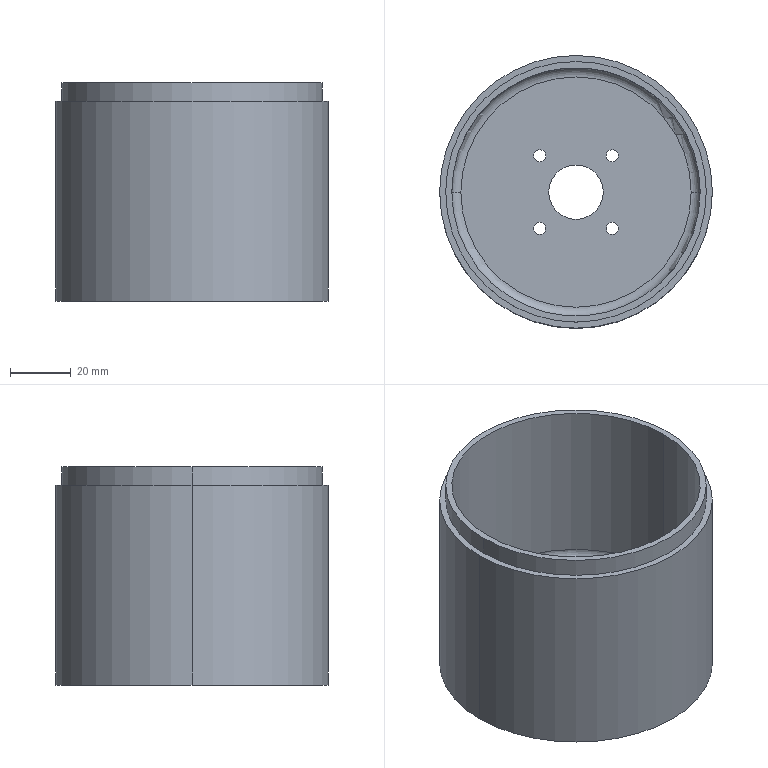Component | SolidWorks | g11-1 | 1 solid | 30 faces | box 90 x 90 x 72 mm | volume 88290 mm3 | cylinder 20 | plane 6 | torus 4 | commonest cylinder face diameters 4 x8 86 x4 82 x4 18 x2 90 x2
STEP:
#1=CARTESIAN_POINT('',(1.066,-0.06694,2.598));
#2=VERTEX_POINT('',#1);
#3=CARTESIAN_POINT('',(-2.32,-0.06694,2.598));
#4=VERTEX_POINT('',#3);
#5=CARTESIAN_POINT('',(-0.6271,-0.06694,2.598));
#6=DIRECTION('',(0.,0.,-1.));
#7=DIRECTION('',(-1.,0.,0.));
#8=AXIS2_PLACEMENT_3D('',#5,#6,#7);
#9=CIRCLE('',#8,1.693);
#10=EDGE_CURVE('',#2,#4,#9,.T.);
#11=ORIENTED_EDGE('',*,*,#10,.F.);
#12=CARTESIAN_POINT('',(1.066,-0.06694,2.441));
#13=VERTEX_POINT('',#12);
#14=CARTESIAN_POINT('',(1.066,-0.06694,2.165));
#15=DIRECTION('',(0.,0.,-1.));
#16=VECTOR('',#15,39.37);
#17=LINE('',#14,#16);
#18=EDGE_CURVE('',#2,#13,#17,.T.);
#19=ORIENTED_EDGE('',*,*,#18,.T.);
#20=CARTESIAN_POINT('',(-2.32,-0.06694,2.441));
#21=VERTEX_POINT('',#20);
#22=CARTESIAN_POINT('',(-0.6271,-0.06694,2.441));
#23=DIRECTION('',(0.,0.,-1.));
#24=DIRECTION('',(-1.,0.,0.));
#25=AXIS2_PLACEMENT_3D('',#22,#23,#24);
#26=CIRCLE('',#25,1.693);
#27=EDGE_CURVE('',#13,#21,#26,.T.);
#28=ORIENTED_EDGE('',*,*,#27,.T.);
#29=CARTESIAN_POINT('',(-2.32,-0.06694,2.165));
#30=DIRECTION('',(0.,0.,-1.));
#31=VECTOR('',#30,39.37);
#32=LINE('',#29,#31);
#33=EDGE_CURVE('',#4,#21,#32,.T.);
#34=ORIENTED_EDGE('',*,*,#33,.F.);
#35=EDGE_LOOP('',(#11,#19,#28,#34));
#36=FACE_OUTER_BOUND('',#35,.T.);
#37=CARTESIAN_POINT('',(-0.6271,-0.06694,2.165));
#38=DIRECTION('',(0.,0.,-1.));
#39=DIRECTION('',(-1.,0.,0.));
#40=AXIS2_PLACEMENT_3D('',#37,#38,#39);
#41=CYLINDRICAL_SURFACE('',#40,1.693);
#42=ADVANCED_FACE('',(#36),#41,.F.);
#43=CARTESIAN_POINT('',(-1.178,0.4055,2.992));
#44=VERTEX_POINT('',#43);
#45=CARTESIAN_POINT('',(-1.021,0.4055,2.992));
#46=VERTEX_POINT('',#45);
#47=CARTESIAN_POINT('',(-1.1,0.4055,2.992));
#48=DIRECTION('',(0.,0.,1.));
#49=DIRECTION('',(1.,0.,0.));
#50=AXIS2_PLACEMENT_3D('',#47,#48,#49);
#51=CIRCLE('',#50,0.07874);
#52=EDGE_CURVE('',#44,#46,#51,.T.);
#53=ORIENTED_EDGE('',*,*,#52,.T.);
#54=CARTESIAN_POINT('',(-1.021,0.4055,2.874));
#55=VERTEX_POINT('',#54);
#56=CARTESIAN_POINT('',(-1.021,0.4055,3.268));
#57=DIRECTION('',(0.,0.,-1.));
#58=VECTOR('',#57,39.37);
#59=LINE('',#56,#58);
#60=EDGE_CURVE('',#46,#55,#59,.T.);
#61=ORIENTED_EDGE('',*,*,#60,.T.);
#62=CARTESIAN_POINT('',(-1.178,0.4055,2.874));
#63=VERTEX_POINT('',#62);
#64=CARTESIAN_POINT('',(-1.1,0.4055,2.874));
#65=DIRECTION('',(0.,0.,-1.));
#66=DIRECTION('',(-1.,0.,0.));
#67=AXIS2_PLACEMENT_3D('',#64,#65,#66);
#68=CIRCLE('',#67,0.07874);
#69=EDGE_CURVE('',#55,#63,#68,.T.);
#70=ORIENTED_EDGE('',*,*,#69,.T.);
#71=CARTESIAN_POINT('',(-1.178,0.4055,3.268));
#72=DIRECTION('',(0.,0.,-1.));
#73=VECTOR('',#72,39.37);
#74=LINE('',#71,#73);
#75=EDGE_CURVE('',#44,#63,#74,.T.);
#76=ORIENTED_EDGE('',*,*,#75,.F.);
#77=EDGE_LOOP('',(#53,#61,#70,#76));
#78=FACE_OUTER_BOUND('',#77,.T.);
#79=CARTESIAN_POINT('',(-1.1,0.4055,3.268));
#80=DIRECTION('',(0.,0.,-1.));
#81=DIRECTION('',(-1.,0.,0.));
#82=AXIS2_PLACEMENT_3D('',#79,#80,#81);
#83=CYLINDRICAL_SURFACE('',#82,0.07874);
#84=ADVANCED_FACE('',(#78),#83,.F.);
#85=CARTESIAN_POINT('',(-0.2334,0.4055,2.992));
#86=VERTEX_POINT('',#85);
#87=CARTESIAN_POINT('',(-0.07591,0.4055,2.992));
#88=VERTEX_POINT('',#87);
#89=CARTESIAN_POINT('',(-0.1546,0.4055,2.992));
#90=DIRECTION('',(0.,0.,1.));
#91=DIRECTION('',(1.,0.,0.));
#92=AXIS2_PLACEMENT_3D('',#89,#90,#91);
#93=CIRCLE('',#92,0.07874);
#94=EDGE_CURVE('',#86,#88,#93,.T.);
#95=ORIENTED_EDGE('',*,*,#94,.T.);
#96=CARTESIAN_POINT('',(-0.07591,0.4055,2.874));
#97=VERTEX_POINT('',#96);
#98=CARTESIAN_POINT('',(-0.07591,0.4055,3.268));
#99=DIRECTION('',(0.,0.,-1.));
#100=VECTOR('',#99,39.37);
#101=LINE('',#98,#100);
#102=EDGE_CURVE('',#88,#97,#101,.T.);
#103=ORIENTED_EDGE('',*,*,#102,.T.);
#104=CARTESIAN_POINT('',(-0.2334,0.4055,2.874));
#105=VERTEX_POINT('',#104);
#106=CARTESIAN_POINT('',(-0.1546,0.4055,2.874));
#107=DIRECTION('',(0.,0.,-1.));
#108=DIRECTION('',(-1.,0.,0.));
#109=AXIS2_PLACEMENT_3D('',#106,#107,#108);
#110=CIRCLE('',#109,0.07874);
#111=EDGE_CURVE('',#97,#105,#110,.T.);
#112=ORIENTED_EDGE('',*,*,#111,.T.);
#113=CARTESIAN_POINT('',(-0.2334,0.4055,3.268));
#114=DIRECTION('',(0.,0.,-1.));
#115=VECTOR('',#114,39.37);
#116=LINE('',#113,#115);
#117=EDGE_CURVE('',#86,#105,#116,.T.);
#118=ORIENTED_EDGE('',*,*,#117,.F.);
#119=EDGE_LOOP('',(#95,#103,#112,#118));
#120=FACE_OUTER_BOUND('',#119,.T.);
#121=CARTESIAN_POINT('',(-0.1546,0.4055,3.268));
#122=DIRECTION('',(0.,0.,-1.));
#123=DIRECTION('',(-1.,0.,0.));
#124=AXIS2_PLACEMENT_3D('',#121,#122,#123);
#125=CYLINDRICAL_SURFACE('',#124,0.07874);
#126=ADVANCED_FACE('',(#120),#125,.F.);
#127=CARTESIAN_POINT('',(-0.2334,-0.5394,2.992));
#128=VERTEX_POINT('',#127);
#129=CARTESIAN_POINT('',(-0.07591,-0.5394,2.992));
#130=VERTEX_POINT('',#129);
#131=CARTESIAN_POINT('',(-0.1546,-0.5394,2.992));
#132=DIRECTION('',(0.,0.,1.));
#133=DIRECTION('',(1.,0.,0.));
#134=AXIS2_PLACEMENT_3D('',#131,#132,#133);
#135=CIRCLE('',#134,0.07874);
#136=EDGE_CURVE('',#128,#130,#135,.T.);
#137=ORIENTED_EDGE('',*,*,#136,.T.);
#138=CARTESIAN_POINT('',(-0.07591,-0.5394,2.874));
#139=VERTEX_POINT('',#138);
#140=CARTESIAN_POINT('',(-0.07591,-0.5394,3.268));
#141=DIRECTION('',(0.,0.,-1.));
#142=VECTOR('',#141,39.37);
#143=LINE('',#140,#142);
#144=EDGE_CURVE('',#130,#139,#143,.T.);
#145=ORIENTED_EDGE('',*,*,#144,.T.);
#146=CARTESIAN_POINT('',(-0.2334,-0.5394,2.874));
#147=VERTEX_POINT('',#146);
#148=CARTESIAN_POINT('',(-0.1546,-0.5394,2.874));
#149=DIRECTION('',(0.,0.,-1.));
#150=DIRECTION('',(-1.,0.,0.));
#151=AXIS2_PLACEMENT_3D('',#148,#149,#150);
#152=CIRCLE('',#151,0.07874);
#153=EDGE_CURVE('',#139,#147,#152,.T.);
#154=ORIENTED_EDGE('',*,*,#153,.T.);
#155=CARTESIAN_POINT('',(-0.2334,-0.5394,3.268));
#156=DIRECTION('',(0.,0.,-1.));
#157=VECTOR('',#156,39.37);
#158=LINE('',#155,#157);
#159=EDGE_CURVE('',#128,#147,#158,.T.);
#160=ORIENTED_EDGE('',*,*,#159,.F.);
#161=EDGE_LOOP('',(#137,#145,#154,#160));
#162=FACE_OUTER_BOUND('',#161,.T.);
#163=CARTESIAN_POINT('',(-0.1546,-0.5394,3.268));
#164=DIRECTION('',(0.,0.,-1.));
#165=DIRECTION('',(-1.,0.,0.));
#166=AXIS2_PLACEMENT_3D('',#163,#164,#165);
#167=CYLINDRICAL_SURFACE('',#166,0.07874);
#168=ADVANCED_FACE('',(#162),#167,.F.);
#169=CARTESIAN_POINT('',(-1.178,-0.5394,2.992));
#170=VERTEX_POINT('',#169);
#171=CARTESIAN_POINT('',(-1.021,-0.5394,2.992));
#172=VERTEX_POINT('',#171);
#173=CARTESIAN_POINT('',(-1.1,-0.5394,2.992));
#174=DIRECTION('',(0.,0.,1.));
#175=DIRECTION('',(1.,0.,0.));
#176=AXIS2_PLACEMENT_3D('',#173,#174,#175);
#177=CIRCLE('',#176,0.07874);
#178=EDGE_CURVE('',#170,#172,#177,.T.);
#179=ORIENTED_EDGE('',*,*,#178,.T.);
#180=CARTESIAN_POINT('',(-1.021,-0.5394,2.874));
#181=VERTEX_POINT('',#180);
#182=CARTESIAN_POINT('',(-1.021,-0.5394,3.268));
#183=DIRECTION('',(0.,0.,-1.));
#184=VECTOR('',#183,39.37);
#185=LINE('',#182,#184);
#186=EDGE_CURVE('',#172,#181,#185,.T.);
#187=ORIENTED_EDGE('',*,*,#186,.T.);
#188=CARTESIAN_POINT('',(-1.178,-0.5394,2.874));
#189=VERTEX_POINT('',#188);
#190=CARTESIAN_POINT('',(-1.1,-0.5394,2.874));
#191=DIRECTION('',(0.,0.,-1.));
#192=DIRECTION('',(-1.,0.,0.));
#193=AXIS2_PLACEMENT_3D('',#190,#191,#192);
#194=CIRCLE('',#193,0.07874);
#195=EDGE_CURVE('',#181,#189,#194,.T.);
#196=ORIENTED_EDGE('',*,*,#195,.T.);
#197=CARTESIAN_POINT('',(-1.178,-0.5394,3.268));
#198=DIRECTION('',(0.,0.,-1.));
#199=VECTOR('',#198,39.37);
#200=LINE('',#197,#199);
#201=EDGE_CURVE('',#170,#189,#200,.T.);
#202=ORIENTED_EDGE('',*,*,#201,.F.);
#203=EDGE_LOOP('',(#179,#187,#196,#202));
#204=FACE_OUTER_BOUND('',#203,.T.);
#205=CARTESIAN_POINT('',(-1.1,-0.5394,3.268));
#206=DIRECTION('',(0.,0.,-1.));
#207=DIRECTION('',(-1.,0.,0.));
#208=AXIS2_PLACEMENT_3D('',#205,#206,#207);
#209=CYLINDRICAL_SURFACE('',#208,0.07874);
#210=ADVANCED_FACE('',(#204),#209,.F.);
#211=CARTESIAN_POINT('',(0.869,-0.06694,2.874));
#212=VERTEX_POINT('',#211);
#213=CARTESIAN_POINT('',(-2.123,-0.06694,2.874));
#214=VERTEX_POINT('',#213);
#215=CARTESIAN_POINT('',(-0.6271,-0.06694,2.874));
#216=DIRECTION('',(0.,0.,-1.));
#217=DIRECTION('',(-1.,0.,0.));
#218=AXIS2_PLACEMENT_3D('',#215,#216,#217);
#219=CIRCLE('',#218,1.496);
#220=EDGE_CURVE('',#212,#214,#219,.T.);
#221=ORIENTED_EDGE('',*,*,#220,.F.);
#222=CARTESIAN_POINT('',(0.9871,-0.06694,2.756));
#223=VERTEX_POINT('',#222);
#224=CARTESIAN_POINT('',(0.869,-0.06694,2.756));
#225=DIRECTION('',(-0.,1.,0.));
#226=DIRECTION('',(-1.,-0.,0.));
#227=AXIS2_PLACEMENT_3D('',#224,#225,#226);
#228=CIRCLE('',#227,0.1181);
#229=EDGE_CURVE('',#212,#223,#228,.T.);
#230=ORIENTED_EDGE('',*,*,#229,.T.);
#231=CARTESIAN_POINT('',(-2.241,-0.06694,2.756));
#232=VERTEX_POINT('',#231);
#233=CARTESIAN_POINT('',(-0.6271,-0.06694,2.756));
#234=DIRECTION('',(0.,0.,1.));
#235=DIRECTION('',(-1.,0.,0.));
#236=AXIS2_PLACEMENT_3D('',#233,#234,#235);
#237=CIRCLE('',#236,1.614);
#238=EDGE_CURVE('',#232,#223,#237,.T.);
#239=ORIENTED_EDGE('',*,*,#238,.F.);
#240=CARTESIAN_POINT('',(-2.123,-0.06694,2.756));
#241=DIRECTION('',(0.,-1.,0.));
#242=DIRECTION('',(0.,0.,-1.));
#243=AXIS2_PLACEMENT_3D('',#240,#241,#242);
#244=CIRCLE('',#243,0.1181);
#245=EDGE_CURVE('',#214,#232,#244,.T.);
#246=ORIENTED_EDGE('',*,*,#245,.F.);
#247=EDGE_LOOP('',(#221,#230,#239,#246));
#248=FACE_OUTER_BOUND('',#247,.T.);
#249=CARTESIAN_POINT('',(-0.6271,-0.06694,2.756));
#250=DIRECTION('',(0.,0.,-1.));
#251=DIRECTION('',(-1.,0.,0.));
#252=AXIS2_PLACEMENT_3D('',#249,#250,#251);
#253=TOROIDAL_SURFACE('',#252,1.496,0.1181);
#254=ADVANCED_FACE('',(#248),#253,.F.);
#255=CARTESIAN_POINT('',(-2.123,-0.06694,2.992));
#256=VERTEX_POINT('',#255);
#257=CARTESIAN_POINT('',(0.869,-0.06694,2.992));
#258=VERTEX_POINT('',#257);
#259=CARTESIAN_POINT('',(-0.6271,-0.06694,2.992));
#260=DIRECTION('',(0.,0.,1.));
#261=DIRECTION('',(1.,0.,0.));
#262=AXIS2_PLACEMENT_3D('',#259,#260,#261);
#263=CIRCLE('',#262,1.496);
#264=EDGE_CURVE('',#256,#258,#263,.T.);
#265=ORIENTED_EDGE('',*,*,#264,.F.);
#266=CARTESIAN_POINT('',(-2.241,-0.06694,3.11));
#267=VERTEX_POINT('',#266);
#268=CARTESIAN_POINT('',(-2.123,-0.06694,3.11));
#269=DIRECTION('',(0.,1.,0.));
#270=DIRECTION('',(-1.,0.,0.));
#271=AXIS2_PLACEMENT_3D('',#268,#269,#270);
#272=CIRCLE('',#271,0.1181);
#273=EDGE_CURVE('',#256,#267,#272,.T.);
#274=ORIENTED_EDGE('',*,*,#273,.T.);
#275=CARTESIAN_POINT('',(0.9871,-0.06694,3.11));
#276=VERTEX_POINT('',#275);
#277=CARTESIAN_POINT('',(-0.6271,-0.06694,3.11));
#278=DIRECTION('',(0.,0.,-1.));
#279=DIRECTION('',(1.,0.,0.));
#280=AXIS2_PLACEMENT_3D('',#277,#278,#279);
#281=CIRCLE('',#280,1.614);
#282=EDGE_CURVE('',#276,#267,#281,.T.);
#283=ORIENTED_EDGE('',*,*,#282,.F.);
#284=CARTESIAN_POINT('',(0.869,-0.06694,3.11));
#285=DIRECTION('',(0.,-1.,0.));
#286=DIRECTION('',(0.,0.,-1.));
#287=AXIS2_PLACEMENT_3D('',#284,#285,#286);
#288=CIRCLE('',#287,0.1181);
#289=EDGE_CURVE('',#258,#276,#288,.T.);
#290=ORIENTED_EDGE('',*,*,#289,.F.);
#291=EDGE_LOOP('',(#265,#274,#283,#290));
#292=FACE_OUTER_BOUND('',#291,.T.);
#293=CARTESIAN_POINT('',(-0.6271,-0.06694,3.11));
#294=DIRECTION('',(0.,0.,1.));
#295=DIRECTION('',(1.,0.,0.));
#296=AXIS2_PLACEMENT_3D('',#293,#294,#295);
#297=TOROIDAL_SURFACE('',#296,1.496,0.1181);
#298=ADVANCED_FACE('',(#292),#297,.F.);
#299=CARTESIAN_POINT('',(-0.2728,-0.06694,2.992));
#300=VERTEX_POINT('',#299);
#301=CARTESIAN_POINT('',(-0.9814,-0.06694,2.992));
#302=VERTEX_POINT('',#301);
#303=CARTESIAN_POINT('',(-0.6271,-0.06694,2.992));
#304=DIRECTION('',(0.,0.,-1.));
#305=DIRECTION('',(-1.,0.,0.));
#306=AXIS2_PLACEMENT_3D('',#303,#304,#305);
#307=CIRCLE('',#306,0.3543);
#308=EDGE_CURVE('',#300,#302,#307,.T.);
#309=ORIENTED_EDGE('',*,*,#308,.F.);
#310=CARTESIAN_POINT('',(-0.2728,-0.06694,2.874));
#311=VERTEX_POINT('',#310);
#312=CARTESIAN_POINT('',(-0.2728,-0.06694,2.441));
#313=DIRECTION('',(0.,0.,-1.));
#314=VECTOR('',#313,39.37);
#315=LINE('',#312,#314);
#316=EDGE_CURVE('',#300,#311,#315,.T.);
#317=ORIENTED_EDGE('',*,*,#316,.T.);
#318=CARTESIAN_POINT('',(-0.9814,-0.06694,2.874));
#319=VERTEX_POINT('',#318);
#320=CARTESIAN_POINT('',(-0.6271,-0.06694,2.874));
#321=DIRECTION('',(0.,0.,-1.));
#322=DIRECTION('',(-1.,0.,0.));
#323=AXIS2_PLACEMENT_3D('',#320,#321,#322);
#324=CIRCLE('',#323,0.3543);
#325=EDGE_CURVE('',#311,#319,#324,.T.);
#326=ORIENTED_EDGE('',*,*,#325,.T.);
#327=CARTESIAN_POINT('',(-0.9814,-0.06694,2.441));
#328=DIRECTION('',(0.,0.,-1.));
#329=VECTOR('',#328,39.37);
#330=LINE('',#327,#329);
#331=EDGE_CURVE('',#302,#319,#330,.T.);
#332=ORIENTED_EDGE('',*,*,#331,.F.);
#333=EDGE_LOOP('',(#309,#317,#326,#332));
#334=FACE_OUTER_BOUND('',#333,.T.);
#335=CARTESIAN_POINT('',(-0.6271,-0.06694,2.441));
#336=DIRECTION('',(0.,0.,-1.));
#337=DIRECTION('',(-1.,0.,0.));
#338=AXIS2_PLACEMENT_3D('',#335,#336,#337);
#339=CYLINDRICAL_SURFACE('',#338,0.3543);
#340=ADVANCED_FACE('',(#334),#339,.F.);
#341=CARTESIAN_POINT('',(-2.32,-0.06694,5.276));
#342=VERTEX_POINT('',#341);
#343=CARTESIAN_POINT('',(1.066,-0.06694,5.276));
#344=VERTEX_POINT('',#343);
#345=CARTESIAN_POINT('',(-0.6271,-0.06694,5.276));
#346=DIRECTION('',(0.,0.,-1.));
#347=DIRECTION('',(-1.,0.,0.));
#348=AXIS2_PLACEMENT_3D('',#345,#346,#347);
#349=CIRCLE('',#348,1.693);
#350=EDGE_CURVE('',#342,#344,#349,.T.);
#351=ORIENTED_EDGE('',*,*,#350,.T.);
#352=CARTESIAN_POINT('',(1.066,-0.06694,5.039));
#353=VERTEX_POINT('',#352);
#354=CARTESIAN_POINT('',(1.066,-0.06694,5.276));
#355=DIRECTION('',(0.,0.,-1.));
#356=VECTOR('',#355,39.37);
#357=LINE('',#354,#356);
#358=EDGE_CURVE('',#344,#353,#357,.T.);
#359=ORIENTED_EDGE('',*,*,#358,.T.);
#360=CARTESIAN_POINT('',(-2.32,-0.06694,5.039));
#361=VERTEX_POINT('',#360);
#362=CARTESIAN_POINT('',(-0.6271,-0.06694,5.039));
#363=DIRECTION('',(0.,0.,1.));
#364=DIRECTION('',(1.,0.,0.));
#365=AXIS2_PLACEMENT_3D('',#362,#363,#364);
#366=CIRCLE('',#365,1.693);
#367=EDGE_CURVE('',#353,#361,#366,.T.);
#368=ORIENTED_EDGE('',*,*,#367,.T.);
#369=CARTESIAN_POINT('',(-2.32,-0.06694,5.276));
#370=DIRECTION('',(0.,0.,-1.));
#371=VECTOR('',#370,39.37);
#372=LINE('',#369,#371);
#373=EDGE_CURVE('',#342,#361,#372,.T.);
#374=ORIENTED_EDGE('',*,*,#373,.F.);
#375=EDGE_LOOP('',(#351,#359,#368,#374));
#376=FACE_OUTER_BOUND('',#375,.T.);
#377=CARTESIAN_POINT('',(-0.6271,-0.06694,5.276));
#378=DIRECTION('',(0.,0.,-1.));
#379=DIRECTION('',(-1.,0.,0.));
#380=AXIS2_PLACEMENT_3D('',#377,#378,#379);
#381=CYLINDRICAL_SURFACE('',#380,1.693);
#382=ADVANCED_FACE('',(#376),#381,.T.);
#383=ORIENTED_EDGE('',*,*,#238,.T.);
#384=CARTESIAN_POINT('',(0.9871,-0.06694,2.598));
#385=VERTEX_POINT('',#384);
#386=CARTESIAN_POINT('',(0.9871,-0.06694,5.039));
#387=DIRECTION('',(0.,0.,-1.));
#388=VECTOR('',#387,39.37);
#389=LINE('',#386,#388);
#390=EDGE_CURVE('',#223,#385,#389,.T.);
#391=ORIENTED_EDGE('',*,*,#390,.T.);
#392=CARTESIAN_POINT('',(-2.241,-0.06694,2.598));
#393=VERTEX_POINT('',#392);
#394=CARTESIAN_POINT('',(-0.6271,-0.06694,2.598));
#395=DIRECTION('',(0.,0.,1.));
#396=DIRECTION('',(1.,0.,0.));
#397=AXIS2_PLACEMENT_3D('',#394,#395,#396);
#398=CIRCLE('',#397,1.614);
#399=EDGE_CURVE('',#393,#385,#398,.T.);
#400=ORIENTED_EDGE('',*,*,#399,.F.);
#401=CARTESIAN_POINT('',(-2.241,-0.06694,5.039));
#402=DIRECTION('',(0.,0.,-1.));
#403=VECTOR('',#402,39.37);
#404=LINE('',#401,#403);
#405=EDGE_CURVE('',#232,#393,#404,.T.);
#406=ORIENTED_EDGE('',*,*,#405,.F.);
#407=EDGE_LOOP('',(#383,#391,#400,#406));
#408=FACE_OUTER_BOUND('',#407,.T.);
#409=CARTESIAN_POINT('',(-0.6271,-0.06694,5.039));
#410=DIRECTION('',(0.,0.,-1.));
#411=DIRECTION('',(-1.,0.,0.));
#412=AXIS2_PLACEMENT_3D('',#409,#410,#411);
#413=CYLINDRICAL_SURFACE('',#412,1.614);
#414=ADVANCED_FACE('',(#408),#413,.F.);
#415=CARTESIAN_POINT('',(1.145,-0.06694,5.039));
#416=VERTEX_POINT('',#415);
#417=CARTESIAN_POINT('',(-2.399,-0.06694,5.039));
#418=VERTEX_POINT('',#417);
#419=CARTESIAN_POINT('',(-0.6271,-0.06694,5.039));
#420=DIRECTION('',(0.,0.,1.));
#421=DIRECTION('',(1.,0.,0.));
#422=AXIS2_PLACEMENT_3D('',#419,#420,#421);
#423=CIRCLE('',#422,1.772);
#424=EDGE_CURVE('',#416,#418,#423,.T.);
#425=ORIENTED_EDGE('',*,*,#424,.F.);
#426=CARTESIAN_POINT('',(1.145,-0.06694,2.441));
#427=VERTEX_POINT('',#426);
#428=CARTESIAN_POINT('',(1.145,-0.06694,5.039));
#429=DIRECTION('',(0.,0.,-1.));
#430=VECTOR('',#429,39.37);
#431=LINE('',#428,#430);
#432=EDGE_CURVE('',#416,#427,#431,.T.);
#433=ORIENTED_EDGE('',*,*,#432,.T.);
#434=CARTESIAN_POINT('',(-2.399,-0.06694,2.441));
#435=VERTEX_POINT('',#434);
#436=CARTESIAN_POINT('',(-0.6271,-0.06694,2.441));
#437=DIRECTION('',(0.,0.,-1.));
#438=DIRECTION('',(-1.,0.,0.));
#439=AXIS2_PLACEMENT_3D('',#436,#437,#438);
#440=CIRCLE('',#439,1.772);
#441=EDGE_CURVE('',#435,#427,#440,.T.);
#442=ORIENTED_EDGE('',*,*,#441,.F.);
#443=CARTESIAN_POINT('',(-2.399,-0.06694,5.039));
#444=DIRECTION('',(0.,0.,-1.));
#445=VECTOR('',#444,39.37);
#446=LINE('',#443,#445);
#447=EDGE_CURVE('',#418,#435,#446,.T.);
#448=ORIENTED_EDGE('',*,*,#447,.F.);
#449=EDGE_LOOP('',(#425,#433,#442,#448));
#450=FACE_OUTER_BOUND('',#449,.T.);
#451=CARTESIAN_POINT('',(-0.6271,-0.06694,5.039));
#452=DIRECTION('',(0.,0.,-1.));
#453=DIRECTION('',(-1.,0.,0.));
#454=AXIS2_PLACEMENT_3D('',#451,#452,#453);
#455=CYLINDRICAL_SURFACE('',#454,1.772);
#456=ADVANCED_FACE('',(#450),#455,.T.);
#457=CARTESIAN_POINT('',(0.9871,-0.06694,5.276));
#458=VERTEX_POINT('',#457);
#459=CARTESIAN_POINT('',(-2.241,-0.06694,5.276));
#460=VERTEX_POINT('',#459);
#461=CARTESIAN_POINT('',(-0.6271,-0.06694,5.276));
#462=DIRECTION('',(0.,0.,-1.));
#463=DIRECTION('',(-1.,0.,0.));
#464=AXIS2_PLACEMENT_3D('',#461,#462,#463);
#465=CIRCLE('',#464,1.614);
#466=EDGE_CURVE('',#458,#460,#465,.T.);
#467=ORIENTED_EDGE('',*,*,#466,.F.);
#468=CARTESIAN_POINT('',(0.9871,-0.06694,5.039));
#469=DIRECTION('',(0.,0.,-1.));
#470=VECTOR('',#469,39.37);
#471=LINE('',#468,#470);
#472=EDGE_CURVE('',#458,#276,#471,.T.);
#473=ORIENTED_EDGE('',*,*,#472,.T.);
#474=ORIENTED_EDGE('',*,*,#282,.T.);
#475=CARTESIAN_POINT('',(-2.241,-0.06694,5.039));
#476=DIRECTION('',(0.,0.,-1.));
#477=VECTOR('',#476,39.37);
#478=LINE('',#475,#477);
#479=EDGE_CURVE('',#460,#267,#478,.T.);
#480=ORIENTED_EDGE('',*,*,#479,.F.);
#481=EDGE_LOOP('',(#467,#473,#474,#480));
#482=FACE_OUTER_BOUND('',#481,.T.);
#483=CARTESIAN_POINT('',(-0.6271,-0.06694,5.039));
#484=DIRECTION('',(0.,0.,-1.));
#485=DIRECTION('',(-1.,0.,0.));
#486=AXIS2_PLACEMENT_3D('',#483,#484,#485);
#487=CYLINDRICAL_SURFACE('',#486,1.614);
#488=ADVANCED_FACE('',(#482),#487,.F.);
#489=ORIENTED_EDGE('',*,*,#472,.F.);
#490=CARTESIAN_POINT('',(-0.6271,-0.06694,5.276));
#491=DIRECTION('',(0.,0.,-1.));
#492=DIRECTION('',(-1.,0.,0.));
#493=AXIS2_PLACEMENT_3D('',#490,#491,#492);
#494=CIRCLE('',#493,1.614);
#495=EDGE_CURVE('',#460,#458,#494,.T.);
#496=ORIENTED_EDGE('',*,*,#495,.F.);
#497=ORIENTED_EDGE('',*,*,#479,.T.);
#498=CARTESIAN_POINT('',(-0.6271,-0.06694,3.11));
#499=DIRECTION('',(0.,0.,-1.));
#500=DIRECTION('',(1.,0.,0.));
#501=AXIS2_PLACEMENT_3D('',#498,#499,#500);
#502=CIRCLE('',#501,1.614);
#503=EDGE_CURVE('',#267,#276,#502,.T.);
#504=ORIENTED_EDGE('',*,*,#503,.T.);
#505=EDGE_LOOP('',(#489,#496,#497,#504));
#506=FACE_OUTER_BOUND('',#505,.T.);
#507=CARTESIAN_POINT('',(-0.6271,-0.06694,5.039));
#508=DIRECTION('',(0.,0.,-1.));
#509=DIRECTION('',(-1.,0.,0.));
#510=AXIS2_PLACEMENT_3D('',#507,#508,#509);
#511=CYLINDRICAL_SURFACE('',#510,1.614);
#512=ADVANCED_FACE('',(#506),#511,.F.);
#513=CARTESIAN_POINT('',(-0.6271,-0.06694,5.039));
#514=DIRECTION('',(0.,0.,1.));
#515=DIRECTION('',(1.,0.,0.));
#516=AXIS2_PLACEMENT_3D('',#513,#514,#515);
#517=CIRCLE('',#516,1.693);
#518=EDGE_CURVE('',#361,#353,#517,.T.);
#519=ORIENTED_EDGE('',*,*,#518,.F.);
#520=ORIENTED_EDGE('',*,*,#367,.F.);
#521=EDGE_LOOP('',(#519,#520));
#522=FACE_BOUND('',#521,.T.);
#523=CARTESIAN_POINT('',(-0.6271,-0.06694,5.039));
#524=DIRECTION('',(0.,0.,1.));
#525=DIRECTION('',(1.,0.,0.));
#526=AXIS2_PLACEMENT_3D('',#523,#524,#525);
#527=CIRCLE('',#526,1.772);
#528=EDGE_CURVE('',#418,#416,#527,.T.);
#529=ORIENTED_EDGE('',*,*,#528,.T.);
#530=ORIENTED_EDGE('',*,*,#424,.T.);
#531=EDGE_LOOP('',(#529,#530));
#532=FACE_OUTER_BOUND('',#531,.T.);
#533=CARTESIAN_POINT('',(-0.6271,-0.06694,5.039));
#534=DIRECTION('',(0.,0.,1.));
#535=DIRECTION('',(1.,0.,0.));
#536=AXIS2_PLACEMENT_3D('',#533,#534,#535);
#537=PLANE('',#536);
#538=ADVANCED_FACE('',(#522,#532),#537,.T.);
#539=ORIENTED_EDGE('',*,*,#432,.F.);
#540=ORIENTED_EDGE('',*,*,#528,.F.);
#541=ORIENTED_EDGE('',*,*,#447,.T.);
#542=CARTESIAN_POINT('',(-0.6271,-0.06694,2.441));
#543=DIRECTION('',(0.,0.,-1.));
#544=DIRECTION('',(-1.,0.,0.));
#545=AXIS2_PLACEMENT_3D('',#542,#543,#544);
#546=CIRCLE('',#545,1.772);
#547=EDGE_CURVE('',#427,#435,#546,.T.);
#548=ORIENTED_EDGE('',*,*,#547,.F.);
#549=EDGE_LOOP('',(#539,#540,#541,#548));
#550=FACE_OUTER_BOUND('',#549,.T.);
#551=CARTESIAN_POINT('',(-0.6271,-0.06694,5.039));
#552=DIRECTION('',(0.,0.,-1.));
#553=DIRECTION('',(-1.,0.,0.));
#554=AXIS2_PLACEMENT_3D('',#551,#552,#553);
#555=CYLINDRICAL_SURFACE('',#554,1.772);
#556=ADVANCED_FACE('',(#550),#555,.T.);
#557=ORIENTED_EDGE('',*,*,#390,.F.);
#558=CARTESIAN_POINT('',(-0.6271,-0.06694,2.756));
#559=DIRECTION('',(0.,0.,1.));
#560=DIRECTION('',(-1.,0.,0.));
#561=AXIS2_PLACEMENT_3D('',#558,#559,#560);
#562=CIRCLE('',#561,1.614);
#563=EDGE_CURVE('',#223,#232,#562,.T.);
#564=ORIENTED_EDGE('',*,*,#563,.T.);
#565=ORIENTED_EDGE('',*,*,#405,.T.);
#566=CARTESIAN_POINT('',(-0.6271,-0.06694,2.598));
#567=DIRECTION('',(0.,0.,1.));
#568=DIRECTION('',(1.,0.,0.));
#569=AXIS2_PLACEMENT_3D('',#566,#567,#568);
#570=CIRCLE('',#569,1.614);
#571=EDGE_CURVE('',#385,#393,#570,.T.);
#572=ORIENTED_EDGE('',*,*,#571,.F.);
#573=EDGE_LOOP('',(#557,#564,#565,#572));
#574=FACE_OUTER_BOUND('',#573,.T.);
#575=CARTESIAN_POINT('',(-0.6271,-0.06694,5.039));
#576=DIRECTION('',(0.,0.,-1.));
#577=DIRECTION('',(-1.,0.,0.));
#578=AXIS2_PLACEMENT_3D('',#575,#576,#577);
#579=CYLINDRICAL_SURFACE('',#578,1.614);
#580=ADVANCED_FACE('',(#574),#579,.F.);
#581=CARTESIAN_POINT('',(-0.6271,-0.06694,2.441));
#582=DIRECTION('',(0.,0.,-1.));
#583=DIRECTION('',(-1.,0.,0.));
#584=AXIS2_PLACEMENT_3D('',#581,#582,#583);
#585=CIRCLE('',#584,1.693);
#586=EDGE_CURVE('',#21,#13,#585,.T.);
#587=ORIENTED_EDGE('',*,*,#586,.F.);
#588=ORIENTED_EDGE('',*,*,#27,.F.);
#589=EDGE_LOOP('',(#587,#588));
#590=FACE_BOUND('',#589,.T.);
#591=ORIENTED_EDGE('',*,*,#441,.T.);
#592=ORIENTED_EDGE('',*,*,#547,.T.);
#593=EDGE_LOOP('',(#591,#592));
#594=FACE_OUTER_BOUND('',#593,.T.);
#595=CARTESIAN_POINT('',(-0.6271,-0.06694,2.441));
#596=DIRECTION('',(0.,0.,-1.));
#597=DIRECTION('',(-1.,0.,0.));
#598=AXIS2_PLACEMENT_3D('',#595,#596,#597);
#599=PLANE('',#598);
#600=ADVANCED_FACE('',(#590,#594),#599,.T.);
#601=ORIENTED_EDGE('',*,*,#358,.F.);
#602=CARTESIAN_POINT('',(-0.6271,-0.06694,5.276));
#603=DIRECTION('',(0.,0.,-1.));
#604=DIRECTION('',(-1.,0.,0.));
#605=AXIS2_PLACEMENT_3D('',#602,#603,#604);
#606=CIRCLE('',#605,1.693);
#607=EDGE_CURVE('',#344,#342,#606,.T.);
#608=ORIENTED_EDGE('',*,*,#607,.T.);
#609=ORIENTED_EDGE('',*,*,#373,.T.);
#610=ORIENTED_EDGE('',*,*,#518,.T.);
#611=EDGE_LOOP('',(#601,#608,#609,#610));
#612=FACE_OUTER_BOUND('',#611,.T.);
#613=CARTESIAN_POINT('',(-0.6271,-0.06694,5.276));
#614=DIRECTION('',(0.,0.,-1.));
#615=DIRECTION('',(-1.,0.,0.));
#616=AXIS2_PLACEMENT_3D('',#613,#614,#615);
#617=CYLINDRICAL_SURFACE('',#616,1.693);
#618=ADVANCED_FACE('',(#612),#617,.T.);
#619=ORIENTED_EDGE('',*,*,#495,.T.);
#620=ORIENTED_EDGE('',*,*,#466,.T.);
#621=EDGE_LOOP('',(#619,#620));
#622=FACE_BOUND('',#621,.T.);
#623=ORIENTED_EDGE('',*,*,#350,.F.);
#624=ORIENTED_EDGE('',*,*,#607,.F.);
#625=EDGE_LOOP('',(#623,#624));
#626=FACE_OUTER_BOUND('',#625,.T.);
#627=CARTESIAN_POINT('',(-0.6271,-0.06694,5.276));
#628=DIRECTION('',(0.,0.,1.));
#629=DIRECTION('',(-1.,0.,0.));
#630=AXIS2_PLACEMENT_3D('',#627,#628,#629);
#631=PLANE('',#630);
#632=ADVANCED_FACE('',(#622,#626),#631,.T.);
#633=ORIENTED_EDGE('',*,*,#52,.F.);
#634=CARTESIAN_POINT('',(-1.1,0.4055,2.992));
#635=DIRECTION('',(0.,0.,1.));
#636=DIRECTION('',(1.,0.,0.));
#637=AXIS2_PLACEMENT_3D('',#634,#635,#636);
#638=CIRCLE('',#637,0.07874);
#639=EDGE_CURVE('',#46,#44,#638,.T.);
#640=ORIENTED_EDGE('',*,*,#639,.F.);
#641=EDGE_LOOP('',(#633,#640));
#642=FACE_BOUND('',#641,.T.);
#643=ORIENTED_EDGE('',*,*,#94,.F.);
#644=CARTESIAN_POINT('',(-0.1546,0.4055,2.992));
#645=DIRECTION('',(0.,0.,1.));
#646=DIRECTION('',(1.,0.,0.));
#647=AXIS2_PLACEMENT_3D('',#644,#645,#646);
#648=CIRCLE('',#647,0.07874);
#649=EDGE_CURVE('',#88,#86,#648,.T.);
#650=ORIENTED_EDGE('',*,*,#649,.F.);
#651=EDGE_LOOP('',(#643,#650));
#652=FACE_BOUND('',#651,.T.);
#653=ORIENTED_EDGE('',*,*,#136,.F.);
#654=CARTESIAN_POINT('',(-0.1546,-0.5394,2.992));
#655=DIRECTION('',(0.,0.,1.));
#656=DIRECTION('',(1.,0.,0.));
#657=AXIS2_PLACEMENT_3D('',#654,#655,#656);
#658=CIRCLE('',#657,0.07874);
#659=EDGE_CURVE('',#130,#128,#658,.T.);
#660=ORIENTED_EDGE('',*,*,#659,.F.);
#661=EDGE_LOOP('',(#653,#660));
#662=FACE_BOUND('',#661,.T.);
#663=ORIENTED_EDGE('',*,*,#178,.F.);
#664=CARTESIAN_POINT('',(-1.1,-0.5394,2.992));
#665=DIRECTION('',(0.,0.,1.));
#666=DIRECTION('',(1.,0.,0.));
#667=AXIS2_PLACEMENT_3D('',#664,#665,#666);
#668=CIRCLE('',#667,0.07874);
#669=EDGE_CURVE('',#172,#170,#668,.T.);
#670=ORIENTED_EDGE('',*,*,#669,.F.);
#671=EDGE_LOOP('',(#663,#670));
#672=FACE_BOUND('',#671,.T.);
#673=CARTESIAN_POINT('',(-0.6271,-0.06694,2.992));
#674=DIRECTION('',(0.,0.,1.));
#675=DIRECTION('',(1.,0.,0.));
#676=AXIS2_PLACEMENT_3D('',#673,#674,#675);
#677=CIRCLE('',#676,1.496);
#678=EDGE_CURVE('',#258,#256,#677,.T.);
#679=ORIENTED_EDGE('',*,*,#678,.T.);
#680=ORIENTED_EDGE('',*,*,#264,.T.);
#681=EDGE_LOOP('',(#679,#680));
#682=FACE_OUTER_BOUND('',#681,.T.);
#683=CARTESIAN_POINT('',(-0.6271,-0.06694,2.992));
#684=DIRECTION('',(0.,0.,-1.));
#685=DIRECTION('',(-1.,0.,0.));
#686=AXIS2_PLACEMENT_3D('',#683,#684,#685);
#687=CIRCLE('',#686,0.3543);
#688=EDGE_CURVE('',#302,#300,#687,.T.);
#689=ORIENTED_EDGE('',*,*,#688,.T.);
#690=ORIENTED_EDGE('',*,*,#308,.T.);
#691=EDGE_LOOP('',(#689,#690));
#692=FACE_BOUND('',#691,.T.);
#693=CARTESIAN_POINT('',(-2.399,-0.06694,2.992));
#694=DIRECTION('',(0.,0.,1.));
#695=DIRECTION('',(1.,0.,0.));
#696=AXIS2_PLACEMENT_3D('',#693,#694,#695);
#697=PLANE('',#696);
#698=ADVANCED_FACE('',(#642,#652,#662,#672,#682,#692),#697,.T.);
#699=ORIENTED_EDGE('',*,*,#316,.F.);
#700=ORIENTED_EDGE('',*,*,#688,.F.);
#701=ORIENTED_EDGE('',*,*,#331,.T.);
#702=CARTESIAN_POINT('',(-0.6271,-0.06694,2.874));
#703=DIRECTION('',(0.,0.,-1.));
#704=DIRECTION('',(-1.,0.,0.));
#705=AXIS2_PLACEMENT_3D('',#702,#703,#704);
#706=CIRCLE('',#705,0.3543);
#707=EDGE_CURVE('',#319,#311,#706,.T.);
#708=ORIENTED_EDGE('',*,*,#707,.T.);
#709=EDGE_LOOP('',(#699,#700,#701,#708));
#710=FACE_OUTER_BOUND('',#709,.T.);
#711=CARTESIAN_POINT('',(-0.6271,-0.06694,2.441));
#712=DIRECTION('',(0.,0.,-1.));
#713=DIRECTION('',(-1.,0.,0.));
#714=AXIS2_PLACEMENT_3D('',#711,#712,#713);
#715=CYLINDRICAL_SURFACE('',#714,0.3543);
#716=ADVANCED_FACE('',(#710),#715,.F.);
#717=CARTESIAN_POINT('',(-1.1,0.4055,2.874));
#718=DIRECTION('',(0.,0.,-1.));
#719=DIRECTION('',(-1.,0.,0.));
#720=AXIS2_PLACEMENT_3D('',#717,#718,#719);
#721=CIRCLE('',#720,0.07874);
#722=EDGE_CURVE('',#63,#55,#721,.T.);
#723=ORIENTED_EDGE('',*,*,#722,.F.);
#724=ORIENTED_EDGE('',*,*,#69,.F.);
#725=EDGE_LOOP('',(#723,#724));
#726=FACE_BOUND('',#725,.T.);
#727=CARTESIAN_POINT('',(-0.1546,0.4055,2.874));
#728=DIRECTION('',(0.,0.,-1.));
#729=DIRECTION('',(-1.,0.,0.));
#730=AXIS2_PLACEMENT_3D('',#727,#728,#729);
#731=CIRCLE('',#730,0.07874);
#732=EDGE_CURVE('',#105,#97,#731,.T.);
#733=ORIENTED_EDGE('',*,*,#732,.F.);
#734=ORIENTED_EDGE('',*,*,#111,.F.);
#735=EDGE_LOOP('',(#733,#734));
#736=FACE_BOUND('',#735,.T.);
#737=CARTESIAN_POINT('',(-0.1546,-0.5394,2.874));
#738=DIRECTION('',(0.,0.,-1.));
#739=DIRECTION('',(-1.,0.,0.));
#740=AXIS2_PLACEMENT_3D('',#737,#738,#739);
#741=CIRCLE('',#740,0.07874);
#742=EDGE_CURVE('',#147,#139,#741,.T.);
#743=ORIENTED_EDGE('',*,*,#742,.F.);
#744=ORIENTED_EDGE('',*,*,#153,.F.);
#745=EDGE_LOOP('',(#743,#744));
#746=FACE_BOUND('',#745,.T.);
#747=CARTESIAN_POINT('',(-1.1,-0.5394,2.874));
#748=DIRECTION('',(0.,0.,-1.));
#749=DIRECTION('',(-1.,0.,0.));
#750=AXIS2_PLACEMENT_3D('',#747,#748,#749);
#751=CIRCLE('',#750,0.07874);
#752=EDGE_CURVE('',#189,#181,#751,.T.);
#753=ORIENTED_EDGE('',*,*,#752,.F.);
#754=ORIENTED_EDGE('',*,*,#195,.F.);
#755=EDGE_LOOP('',(#753,#754));
#756=FACE_BOUND('',#755,.T.);
#757=CARTESIAN_POINT('',(-0.6271,-0.06694,2.874));
#758=DIRECTION('',(0.,0.,-1.));
#759=DIRECTION('',(-1.,0.,0.));
#760=AXIS2_PLACEMENT_3D('',#757,#758,#759);
#761=CIRCLE('',#760,1.496);
#762=EDGE_CURVE('',#214,#212,#761,.T.);
#763=ORIENTED_EDGE('',*,*,#762,.T.);
#764=ORIENTED_EDGE('',*,*,#220,.T.);
#765=EDGE_LOOP('',(#763,#764));
#766=FACE_OUTER_BOUND('',#765,.T.);
#767=ORIENTED_EDGE('',*,*,#707,.F.);
#768=ORIENTED_EDGE('',*,*,#325,.F.);
#769=EDGE_LOOP('',(#767,#768));
#770=FACE_BOUND('',#769,.T.);
#771=CARTESIAN_POINT('',(-2.399,-0.06694,2.874));
#772=DIRECTION('',(0.,0.,-1.));
#773=DIRECTION('',(-1.,0.,0.));
#774=AXIS2_PLACEMENT_3D('',#771,#772,#773);
#775=PLANE('',#774);
#776=ADVANCED_FACE('',(#726,#736,#746,#756,#766,#770),#775,.T.);
#777=ORIENTED_EDGE('',*,*,#273,.F.);
#778=ORIENTED_EDGE('',*,*,#678,.F.);
#779=ORIENTED_EDGE('',*,*,#289,.T.);
#780=ORIENTED_EDGE('',*,*,#503,.F.);
#781=EDGE_LOOP('',(#777,#778,#779,#780));
#782=FACE_OUTER_BOUND('',#781,.T.);
#783=CARTESIAN_POINT('',(-0.6271,-0.06694,3.11));
#784=DIRECTION('',(0.,0.,1.));
#785=DIRECTION('',(1.,0.,0.));
#786=AXIS2_PLACEMENT_3D('',#783,#784,#785);
#787=TOROIDAL_SURFACE('',#786,1.496,0.1181);
#788=ADVANCED_FACE('',(#782),#787,.F.);
#789=ORIENTED_EDGE('',*,*,#229,.F.);
#790=ORIENTED_EDGE('',*,*,#762,.F.);
#791=ORIENTED_EDGE('',*,*,#245,.T.);
#792=ORIENTED_EDGE('',*,*,#563,.F.);
#793=EDGE_LOOP('',(#789,#790,#791,#792));
#794=FACE_OUTER_BOUND('',#793,.T.);
#795=CARTESIAN_POINT('',(-0.6271,-0.06694,2.756));
#796=DIRECTION('',(0.,0.,-1.));
#797=DIRECTION('',(-1.,0.,0.));
#798=AXIS2_PLACEMENT_3D('',#795,#796,#797);
#799=TOROIDAL_SURFACE('',#798,1.496,0.1181);
#800=ADVANCED_FACE('',(#794),#799,.F.);
#801=ORIENTED_EDGE('',*,*,#186,.F.);
#802=ORIENTED_EDGE('',*,*,#669,.T.);
#803=ORIENTED_EDGE('',*,*,#201,.T.);
#804=ORIENTED_EDGE('',*,*,#752,.T.);
#805=EDGE_LOOP('',(#801,#802,#803,#804));
#806=FACE_OUTER_BOUND('',#805,.T.);
#807=CARTESIAN_POINT('',(-1.1,-0.5394,3.268));
#808=DIRECTION('',(0.,0.,-1.));
#809=DIRECTION('',(-1.,0.,0.));
#810=AXIS2_PLACEMENT_3D('',#807,#808,#809);
#811=CYLINDRICAL_SURFACE('',#810,0.07874);
#812=ADVANCED_FACE('',(#806),#811,.F.);
#813=ORIENTED_EDGE('',*,*,#144,.F.);
#814=ORIENTED_EDGE('',*,*,#659,.T.);
#815=ORIENTED_EDGE('',*,*,#159,.T.);
#816=ORIENTED_EDGE('',*,*,#742,.T.);
#817=EDGE_LOOP('',(#813,#814,#815,#816));
#818=FACE_OUTER_BOUND('',#817,.T.);
#819=CARTESIAN_POINT('',(-0.1546,-0.5394,3.268));
#820=DIRECTION('',(0.,0.,-1.));
#821=DIRECTION('',(-1.,0.,0.));
#822=AXIS2_PLACEMENT_3D('',#819,#820,#821);
#823=CYLINDRICAL_SURFACE('',#822,0.07874);
#824=ADVANCED_FACE('',(#818),#823,.F.);
#825=ORIENTED_EDGE('',*,*,#102,.F.);
#826=ORIENTED_EDGE('',*,*,#649,.T.);
#827=ORIENTED_EDGE('',*,*,#117,.T.);
#828=ORIENTED_EDGE('',*,*,#732,.T.);
#829=EDGE_LOOP('',(#825,#826,#827,#828));
#830=FACE_OUTER_BOUND('',#829,.T.);
#831=CARTESIAN_POINT('',(-0.1546,0.4055,3.268));
#832=DIRECTION('',(0.,0.,-1.));
#833=DIRECTION('',(-1.,0.,0.));
#834=AXIS2_PLACEMENT_3D('',#831,#832,#833);
#835=CYLINDRICAL_SURFACE('',#834,0.07874);
#836=ADVANCED_FACE('',(#830),#835,.F.);
#837=ORIENTED_EDGE('',*,*,#60,.F.);
#838=ORIENTED_EDGE('',*,*,#639,.T.);
#839=ORIENTED_EDGE('',*,*,#75,.T.);
#840=ORIENTED_EDGE('',*,*,#722,.T.);
#841=EDGE_LOOP('',(#837,#838,#839,#840));
#842=FACE_OUTER_BOUND('',#841,.T.);
#843=CARTESIAN_POINT('',(-1.1,0.4055,3.268));
#844=DIRECTION('',(0.,0.,-1.));
#845=DIRECTION('',(-1.,0.,0.));
#846=AXIS2_PLACEMENT_3D('',#843,#844,#845);
#847=CYLINDRICAL_SURFACE('',#846,0.07874);
#848=ADVANCED_FACE('',(#842),#847,.F.);
#849=ORIENTED_EDGE('',*,*,#399,.T.);
#850=ORIENTED_EDGE('',*,*,#571,.T.);
#851=EDGE_LOOP('',(#849,#850));
#852=FACE_BOUND('',#851,.T.);
#853=CARTESIAN_POINT('',(-0.6271,-0.06694,2.598));
#854=DIRECTION('',(0.,0.,-1.));
#855=DIRECTION('',(-1.,0.,0.));
#856=AXIS2_PLACEMENT_3D('',#853,#854,#855);
#857=CIRCLE('',#856,1.693);
#858=EDGE_CURVE('',#4,#2,#857,.T.);
#859=ORIENTED_EDGE('',*,*,#858,.T.);
#860=ORIENTED_EDGE('',*,*,#10,.T.);
#861=EDGE_LOOP('',(#859,#860));
#862=FACE_OUTER_BOUND('',#861,.T.);
#863=CARTESIAN_POINT('',(-0.6271,1.626,2.598));
#864=DIRECTION('',(0.,0.,1.));
#865=DIRECTION('',(1.,0.,0.));
#866=AXIS2_PLACEMENT_3D('',#863,#864,#865);
#867=PLANE('',#866);
#868=ADVANCED_FACE('',(#852,#862),#867,.F.);
#869=ORIENTED_EDGE('',*,*,#18,.F.);
#870=ORIENTED_EDGE('',*,*,#858,.F.);
#871=ORIENTED_EDGE('',*,*,#33,.T.);
#872=ORIENTED_EDGE('',*,*,#586,.T.);
#873=EDGE_LOOP('',(#869,#870,#871,#872));
#874=FACE_OUTER_BOUND('',#873,.T.);
#875=CARTESIAN_POINT('',(-0.6271,-0.06694,2.165));
#876=DIRECTION('',(0.,0.,-1.));
#877=DIRECTION('',(-1.,0.,0.));
#878=AXIS2_PLACEMENT_3D('',#875,#876,#877);
#879=CYLINDRICAL_SURFACE('',#878,1.693);
#880=ADVANCED_FACE('',(#874),#879,.F.);
#881=CLOSED_SHELL('',(#42,#84,#126,#168,#210,#254,#298,#340,#382,#414,#456,#488,#512,#538,#556,#580,#600,#618,#632,#698,#716,#776,#788,#800,#812,#824,#836,#848,#868,#880));
#882=MANIFOLD_SOLID_BREP('',#881);
#883=CARTESIAN_POINT('',(0.,0.,0.));
#884=DIRECTION('',(0.,0.,1.));
#885=DIRECTION('',(1.,0.,0.));
#886=AXIS2_PLACEMENT_3D('',#883,#884,#885);
#887=(LENGTH_UNIT()NAMED_UNIT(*)SI_UNIT($,.METRE.));
#888=LENGTH_MEASURE_WITH_UNIT(LENGTH_MEASURE(0.0254),#887);
#889=DIMENSIONAL_EXPONENTS(1.,0.,0.,0.,0.,0.,0.);
#890=(CONVERSION_BASED_UNIT('',#888)LENGTH_UNIT()NAMED_UNIT(#889));
#891=UNCERTAINTY_MEASURE_WITH_UNIT(LENGTH_MEASURE(0.00001),#890,'','');
#892=(NAMED_UNIT(*)PLANE_ANGLE_UNIT()SI_UNIT($,.RADIAN.));
#893=(NAMED_UNIT(*)SI_UNIT($,.STERADIAN.)SOLID_ANGLE_UNIT());
#894=(GEOMETRIC_REPRESENTATION_CONTEXT(3)GLOBAL_UNCERTAINTY_ASSIGNED_CONTEXT((#891))GLOBAL_UNIT_ASSIGNED_CONTEXT((#890,#892,#893))REPRESENTATION_CONTEXT('',''));
#895=ADVANCED_BREP_SHAPE_REPRESENTATION('',(#882,#886),#894);
#896=COLOUR_RGB('',0.7922,0.8196,0.9333);
#897=FILL_AREA_STYLE_COLOUR('',#896);
#898=FILL_AREA_STYLE('',(#897));
#899=SURFACE_STYLE_FILL_AREA(#898);
#900=SURFACE_SIDE_STYLE('',(#899));
#901=SURFACE_STYLE_USAGE(.BOTH.,#900);
#902=PRESENTATION_STYLE_ASSIGNMENT((#901));
#903=STYLED_ITEM('',(#902),#882);
#904=(LENGTH_UNIT()NAMED_UNIT(*)SI_UNIT($,.METRE.));
#905=LENGTH_MEASURE_WITH_UNIT(LENGTH_MEASURE(0.0254),#904);
#906=DIMENSIONAL_EXPONENTS(1.,0.,0.,0.,0.,0.,0.);
#907=(CONVERSION_BASED_UNIT('',#905)LENGTH_UNIT()NAMED_UNIT(#906));
#908=UNCERTAINTY_MEASURE_WITH_UNIT(LENGTH_MEASURE(0.00001),#907,'','');
#909=(NAMED_UNIT(*)PLANE_ANGLE_UNIT()SI_UNIT($,.RADIAN.));
#910=(NAMED_UNIT(*)SI_UNIT($,.STERADIAN.)SOLID_ANGLE_UNIT());
#911=(GEOMETRIC_REPRESENTATION_CONTEXT(3)GLOBAL_UNCERTAINTY_ASSIGNED_CONTEXT((#908))GLOBAL_UNIT_ASSIGNED_CONTEXT((#907,#909,#910))REPRESENTATION_CONTEXT('',''));
#912=MECHANICAL_DESIGN_GEOMETRIC_PRESENTATION_REPRESENTATION('',(#903),#911);
#913=PRESENTATION_LAYER_ASSIGNMENT('','',(#903));